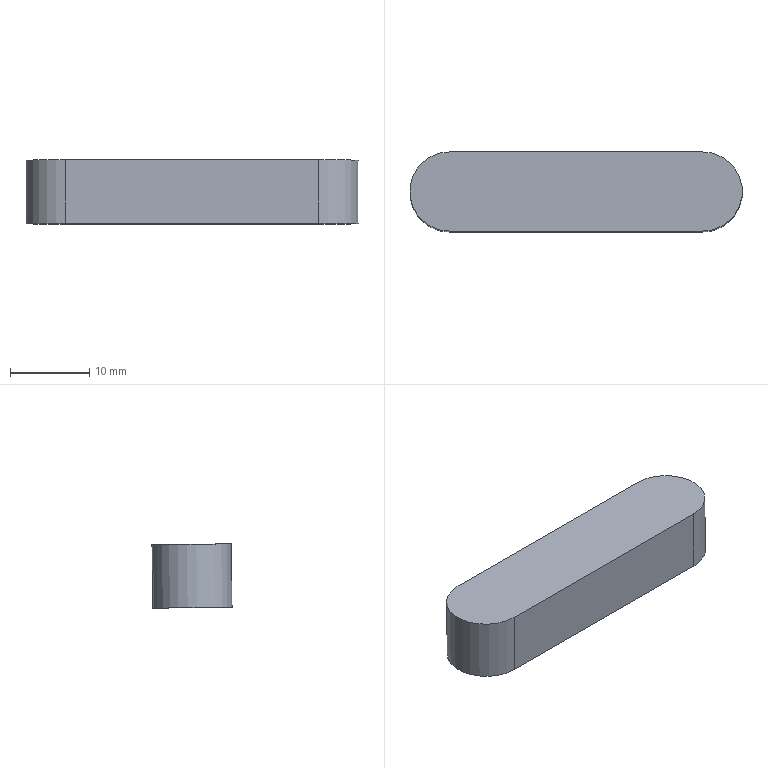Component | SolidWorks | Key1-1 | 1 solid | 6 faces | box 42 x 10.11 x 8.14 mm | volume 3188 mm3 | plane 4 | cylinder 2 | commonest cylinder face diameters 10 x2
build123d program:
from build123d import *

# Parameters (mm, degrees)
BOSS_EXTRUDE1_DEPTH = 8


with BuildPart() as part:
    # Sketch1 → Boss-Extrude1 (new body)
    with BuildSketch(Plane(origin=(0, 0, 0), x_dir=(1, 0, 0), z_dir=(0, 1, 0))):
        with BuildLine():
            Line((-16, 5), (16, 5))
            ThreePointArc((16, 5), (21, 0), (16, -5))
            Line((16, -5), (-16, -5))
            ThreePointArc((-16, -5), (-21, 0), (-16, 5))
        make_face()
    extrude(amount=BOSS_EXTRUDE1_DEPTH)


solid = part.part

# Placed as in the assembly
solid = solid.moved(Location((143.571, -8.995, -195.997), (89.199, 0, 0)))
STEP:
#1=CARTESIAN_POINT('',(6.282,-0.551,-7.714));
#2=VERTEX_POINT('',#1);
#3=CARTESIAN_POINT('',(6.282,-0.1573,-7.719));
#4=VERTEX_POINT('',#3);
#5=CARTESIAN_POINT('',(6.282,-0.3541,-7.716));
#6=DIRECTION('',(-0.,0.01398,0.9999));
#7=DIRECTION('',(0.,0.9999,-0.01398));
#8=AXIS2_PLACEMENT_3D('',#5,#6,#7);
#9=CIRCLE('',#8,0.1969);
#10=EDGE_CURVE('',#2,#4,#9,.T.);
#11=ORIENTED_EDGE('',*,*,#10,.T.);
#12=CARTESIAN_POINT('',(6.282,-0.1529,-7.404));
#13=VERTEX_POINT('',#12);
#14=CARTESIAN_POINT('',(6.282,-0.1529,-7.404));
#15=DIRECTION('',(0.,-0.01398,-0.9999));
#16=VECTOR('',#15,39.37);
#17=LINE('',#14,#16);
#18=EDGE_CURVE('',#13,#4,#17,.T.);
#19=ORIENTED_EDGE('',*,*,#18,.F.);
#20=CARTESIAN_POINT('',(6.282,-0.5466,-7.399));
#21=VERTEX_POINT('',#20);
#22=CARTESIAN_POINT('',(6.282,-0.3497,-7.401));
#23=DIRECTION('',(-0.,0.01398,0.9999));
#24=DIRECTION('',(0.,0.9999,-0.01398));
#25=AXIS2_PLACEMENT_3D('',#22,#23,#24);
#26=CIRCLE('',#25,0.1969);
#27=EDGE_CURVE('',#21,#13,#26,.T.);
#28=ORIENTED_EDGE('',*,*,#27,.F.);
#29=CARTESIAN_POINT('',(6.282,-0.5466,-7.399));
#30=DIRECTION('',(0.,-0.01398,-0.9999));
#31=VECTOR('',#30,39.37);
#32=LINE('',#29,#31);
#33=EDGE_CURVE('',#21,#2,#32,.T.);
#34=ORIENTED_EDGE('',*,*,#33,.T.);
#35=EDGE_LOOP('',(#11,#19,#28,#34));
#36=FACE_OUTER_BOUND('',#35,.T.);
#37=CARTESIAN_POINT('',(6.282,-0.3497,-7.401));
#38=DIRECTION('',(0.,-0.01398,-0.9999));
#39=DIRECTION('',(0.,-0.9999,0.01398));
#40=AXIS2_PLACEMENT_3D('',#37,#38,#39);
#41=CYLINDRICAL_SURFACE('',#40,0.1969);
#42=ADVANCED_FACE('',(#36),#41,.T.);
#43=CARTESIAN_POINT('',(5.022,-0.1573,-7.719));
#44=VERTEX_POINT('',#43);
#45=CARTESIAN_POINT('',(5.022,-0.1573,-7.719));
#46=DIRECTION('',(-1.,-0.,-0.));
#47=VECTOR('',#46,39.37);
#48=LINE('',#45,#47);
#49=EDGE_CURVE('',#4,#44,#48,.T.);
#50=ORIENTED_EDGE('',*,*,#49,.T.);
#51=CARTESIAN_POINT('',(5.022,-0.1529,-7.404));
#52=VERTEX_POINT('',#51);
#53=CARTESIAN_POINT('',(5.022,-0.1529,-7.404));
#54=DIRECTION('',(0.,-0.01398,-0.9999));
#55=VECTOR('',#54,39.37);
#56=LINE('',#53,#55);
#57=EDGE_CURVE('',#52,#44,#56,.T.);
#58=ORIENTED_EDGE('',*,*,#57,.F.);
#59=CARTESIAN_POINT('',(5.022,-0.1529,-7.404));
#60=DIRECTION('',(-1.,-0.,-0.));
#61=VECTOR('',#60,39.37);
#62=LINE('',#59,#61);
#63=EDGE_CURVE('',#13,#52,#62,.T.);
#64=ORIENTED_EDGE('',*,*,#63,.F.);
#65=ORIENTED_EDGE('',*,*,#18,.T.);
#66=EDGE_LOOP('',(#50,#58,#64,#65));
#67=FACE_OUTER_BOUND('',#66,.T.);
#68=CARTESIAN_POINT('',(5.022,-0.1529,-7.404));
#69=DIRECTION('',(0.,-0.9999,0.01398));
#70=DIRECTION('',(1.,0.,0.));
#71=AXIS2_PLACEMENT_3D('',#68,#69,#70);
#72=PLANE('',#71);
#73=ADVANCED_FACE('',(#67),#72,.F.);
#74=CARTESIAN_POINT('',(5.022,-0.551,-7.714));
#75=VERTEX_POINT('',#74);
#76=CARTESIAN_POINT('',(5.022,-0.3541,-7.716));
#77=DIRECTION('',(-0.,0.01398,0.9999));
#78=DIRECTION('',(0.,-0.9999,0.01398));
#79=AXIS2_PLACEMENT_3D('',#76,#77,#78);
#80=CIRCLE('',#79,0.1969);
#81=EDGE_CURVE('',#44,#75,#80,.T.);
#82=ORIENTED_EDGE('',*,*,#81,.T.);
#83=CARTESIAN_POINT('',(5.022,-0.5466,-7.399));
#84=VERTEX_POINT('',#83);
#85=CARTESIAN_POINT('',(5.022,-0.5466,-7.399));
#86=DIRECTION('',(0.,-0.01398,-0.9999));
#87=VECTOR('',#86,39.37);
#88=LINE('',#85,#87);
#89=EDGE_CURVE('',#84,#75,#88,.T.);
#90=ORIENTED_EDGE('',*,*,#89,.F.);
#91=CARTESIAN_POINT('',(5.022,-0.3497,-7.401));
#92=DIRECTION('',(-0.,0.01398,0.9999));
#93=DIRECTION('',(0.,-0.9999,0.01398));
#94=AXIS2_PLACEMENT_3D('',#91,#92,#93);
#95=CIRCLE('',#94,0.1969);
#96=EDGE_CURVE('',#52,#84,#95,.T.);
#97=ORIENTED_EDGE('',*,*,#96,.F.);
#98=ORIENTED_EDGE('',*,*,#57,.T.);
#99=EDGE_LOOP('',(#82,#90,#97,#98));
#100=FACE_OUTER_BOUND('',#99,.T.);
#101=CARTESIAN_POINT('',(5.022,-0.3497,-7.401));
#102=DIRECTION('',(0.,-0.01398,-0.9999));
#103=DIRECTION('',(0.,-0.9999,0.01398));
#104=AXIS2_PLACEMENT_3D('',#101,#102,#103);
#105=CYLINDRICAL_SURFACE('',#104,0.1969);
#106=ADVANCED_FACE('',(#100),#105,.T.);
#107=CARTESIAN_POINT('',(6.282,-0.551,-7.714));
#108=DIRECTION('',(1.,0.,0.));
#109=VECTOR('',#108,39.37);
#110=LINE('',#107,#109);
#111=EDGE_CURVE('',#75,#2,#110,.T.);
#112=ORIENTED_EDGE('',*,*,#111,.T.);
#113=ORIENTED_EDGE('',*,*,#33,.F.);
#114=CARTESIAN_POINT('',(6.282,-0.5466,-7.399));
#115=DIRECTION('',(1.,0.,0.));
#116=VECTOR('',#115,39.37);
#117=LINE('',#114,#116);
#118=EDGE_CURVE('',#84,#21,#117,.T.);
#119=ORIENTED_EDGE('',*,*,#118,.F.);
#120=ORIENTED_EDGE('',*,*,#89,.T.);
#121=EDGE_LOOP('',(#112,#113,#119,#120));
#122=FACE_OUTER_BOUND('',#121,.T.);
#123=CARTESIAN_POINT('',(6.282,-0.5466,-7.399));
#124=DIRECTION('',(-0.,0.9999,-0.01398));
#125=DIRECTION('',(-1.,-0.,-0.));
#126=AXIS2_PLACEMENT_3D('',#123,#124,#125);
#127=PLANE('',#126);
#128=ADVANCED_FACE('',(#122),#127,.F.);
#129=ORIENTED_EDGE('',*,*,#27,.T.);
#130=ORIENTED_EDGE('',*,*,#63,.T.);
#131=ORIENTED_EDGE('',*,*,#96,.T.);
#132=ORIENTED_EDGE('',*,*,#118,.T.);
#133=EDGE_LOOP('',(#129,#130,#131,#132));
#134=FACE_OUTER_BOUND('',#133,.T.);
#135=CARTESIAN_POINT('',(6.282,-0.3497,-7.401));
#136=DIRECTION('',(-0.,0.01398,0.9999));
#137=DIRECTION('',(-0.,0.9999,-0.01398));
#138=AXIS2_PLACEMENT_3D('',#135,#136,#137);
#139=PLANE('',#138);
#140=ADVANCED_FACE('',(#134),#139,.T.);
#141=ORIENTED_EDGE('',*,*,#10,.F.);
#142=ORIENTED_EDGE('',*,*,#111,.F.);
#143=ORIENTED_EDGE('',*,*,#81,.F.);
#144=ORIENTED_EDGE('',*,*,#49,.F.);
#145=EDGE_LOOP('',(#141,#142,#143,#144));
#146=FACE_OUTER_BOUND('',#145,.T.);
#147=CARTESIAN_POINT('',(6.282,-0.3541,-7.716));
#148=DIRECTION('',(-0.,0.01398,0.9999));
#149=DIRECTION('',(-0.,0.9999,-0.01398));
#150=AXIS2_PLACEMENT_3D('',#147,#148,#149);
#151=PLANE('',#150);
#152=ADVANCED_FACE('',(#146),#151,.F.);
#153=CLOSED_SHELL('',(#42,#73,#106,#128,#140,#152));
#154=MANIFOLD_SOLID_BREP('',#153);
#155=CARTESIAN_POINT('',(0.,0.,0.));
#156=DIRECTION('',(0.,0.,1.));
#157=DIRECTION('',(1.,0.,0.));
#158=AXIS2_PLACEMENT_3D('',#155,#156,#157);
#159=(LENGTH_UNIT()NAMED_UNIT(*)SI_UNIT($,.METRE.));
#160=LENGTH_MEASURE_WITH_UNIT(LENGTH_MEASURE(0.0254),#159);
#161=DIMENSIONAL_EXPONENTS(1.,0.,0.,0.,0.,0.,0.);
#162=(CONVERSION_BASED_UNIT('',#160)LENGTH_UNIT()NAMED_UNIT(#161));
#163=UNCERTAINTY_MEASURE_WITH_UNIT(LENGTH_MEASURE(0.00001),#162,'','');
#164=(NAMED_UNIT(*)PLANE_ANGLE_UNIT()SI_UNIT($,.RADIAN.));
#165=(NAMED_UNIT(*)SI_UNIT($,.STERADIAN.)SOLID_ANGLE_UNIT());
#166=(GEOMETRIC_REPRESENTATION_CONTEXT(3)GLOBAL_UNCERTAINTY_ASSIGNED_CONTEXT((#163))GLOBAL_UNIT_ASSIGNED_CONTEXT((#162,#164,#165))REPRESENTATION_CONTEXT('',''));
#167=ADVANCED_BREP_SHAPE_REPRESENTATION('',(#154,#158),#166);
#168=COLOUR_RGB('',0.7922,0.8196,0.9333);
#169=FILL_AREA_STYLE_COLOUR('',#168);
#170=FILL_AREA_STYLE('',(#169));
#171=SURFACE_STYLE_FILL_AREA(#170);
#172=SURFACE_SIDE_STYLE('',(#171));
#173=SURFACE_STYLE_USAGE(.BOTH.,#172);
#174=PRESENTATION_STYLE_ASSIGNMENT((#173));
#175=STYLED_ITEM('',(#174),#154);
#176=(LENGTH_UNIT()NAMED_UNIT(*)SI_UNIT($,.METRE.));
#177=LENGTH_MEASURE_WITH_UNIT(LENGTH_MEASURE(0.0254),#176);
#178=DIMENSIONAL_EXPONENTS(1.,0.,0.,0.,0.,0.,0.);
#179=(CONVERSION_BASED_UNIT('',#177)LENGTH_UNIT()NAMED_UNIT(#178));
#180=UNCERTAINTY_MEASURE_WITH_UNIT(LENGTH_MEASURE(0.00001),#179,'','');
#181=(NAMED_UNIT(*)PLANE_ANGLE_UNIT()SI_UNIT($,.RADIAN.));
#182=(NAMED_UNIT(*)SI_UNIT($,.STERADIAN.)SOLID_ANGLE_UNIT());
#183=(GEOMETRIC_REPRESENTATION_CONTEXT(3)GLOBAL_UNCERTAINTY_ASSIGNED_CONTEXT((#180))GLOBAL_UNIT_ASSIGNED_CONTEXT((#179,#181,#182))REPRESENTATION_CONTEXT('',''));
#184=MECHANICAL_DESIGN_GEOMETRIC_PRESENTATION_REPRESENTATION('',(#175),#183);
#185=PRESENTATION_LAYER_ASSIGNMENT('','',(#175));